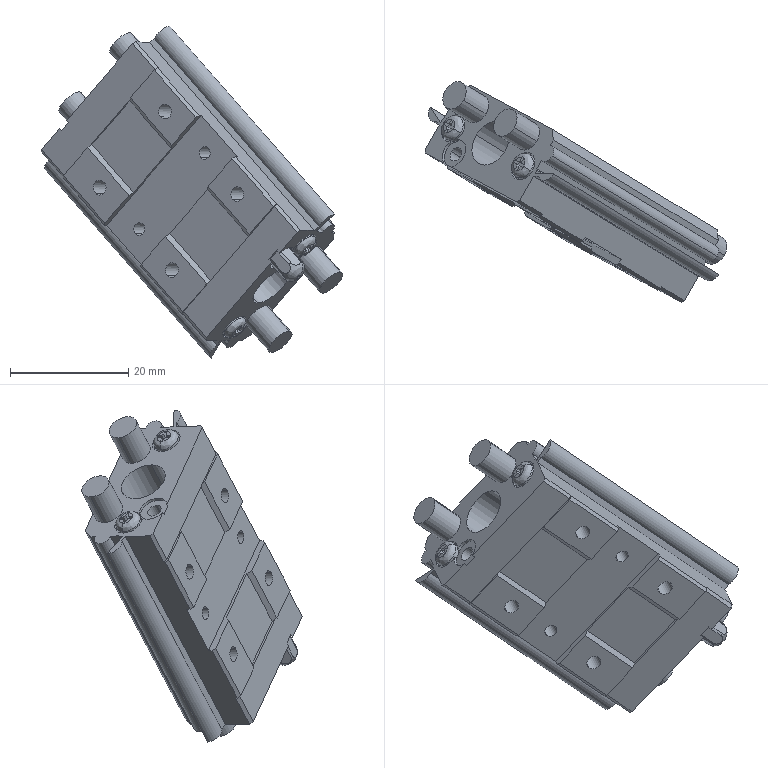Component | SolidWorks | KK40-100A1-F0z0-123-2_KK40-A1_1z0-123-1 | 1 solid | 225 faces | volume 14610 mm3 | plane 154 | cylinder 59 | spline 10 | torus 2 | commonest cylinder face diameters 5 x23 4.4 x15 2.5 x10 2.15 x4 3 x3 8 x2 4 x2